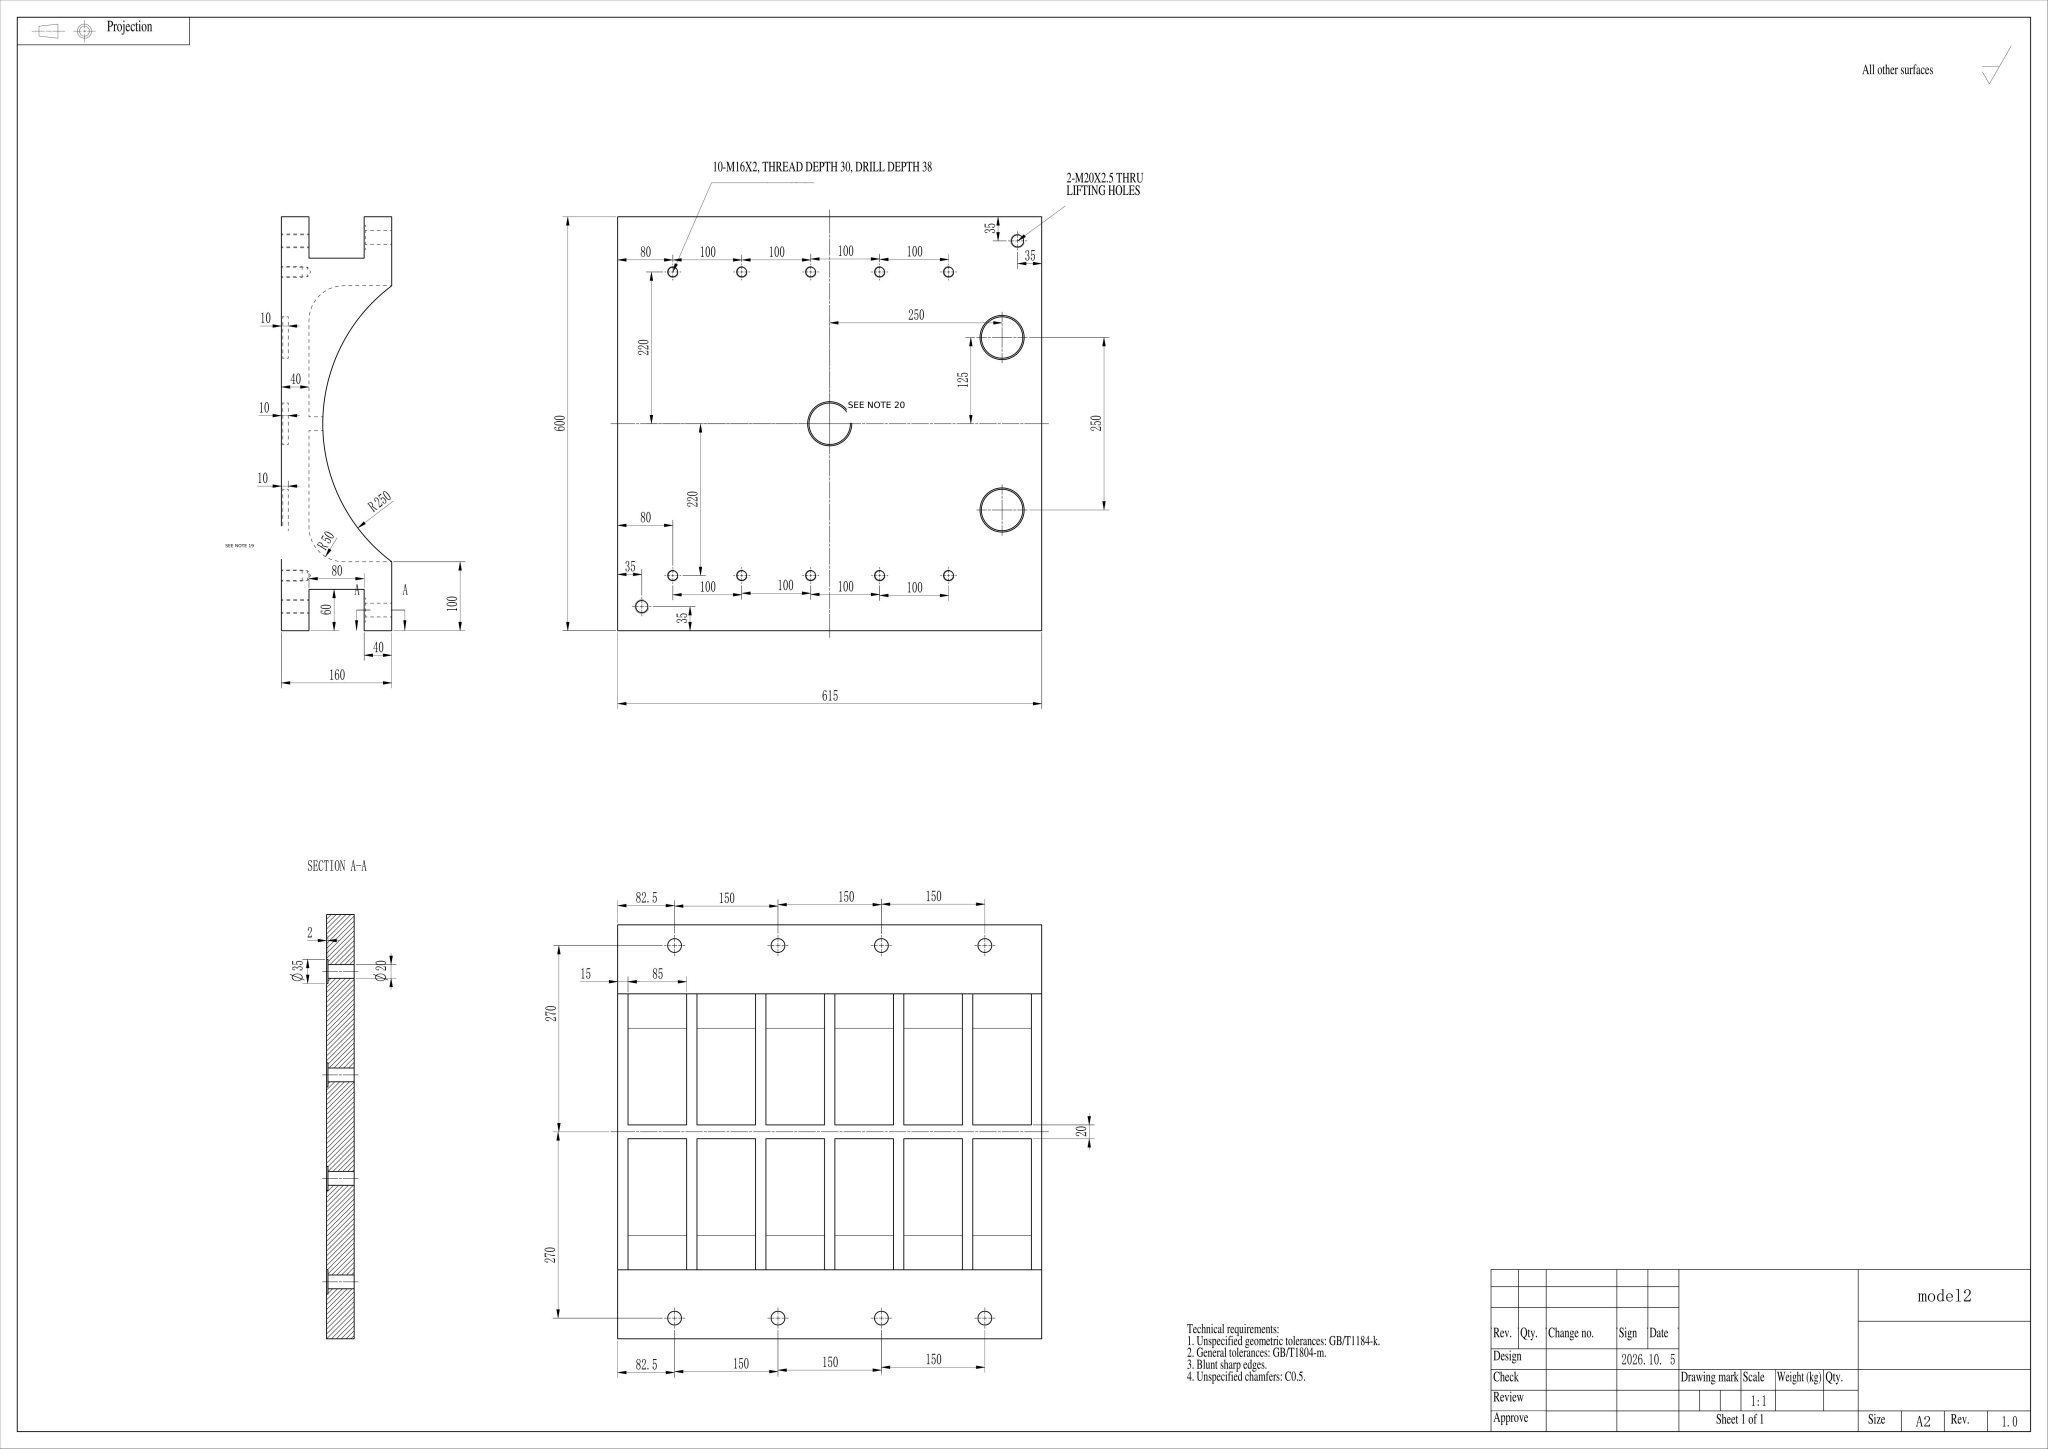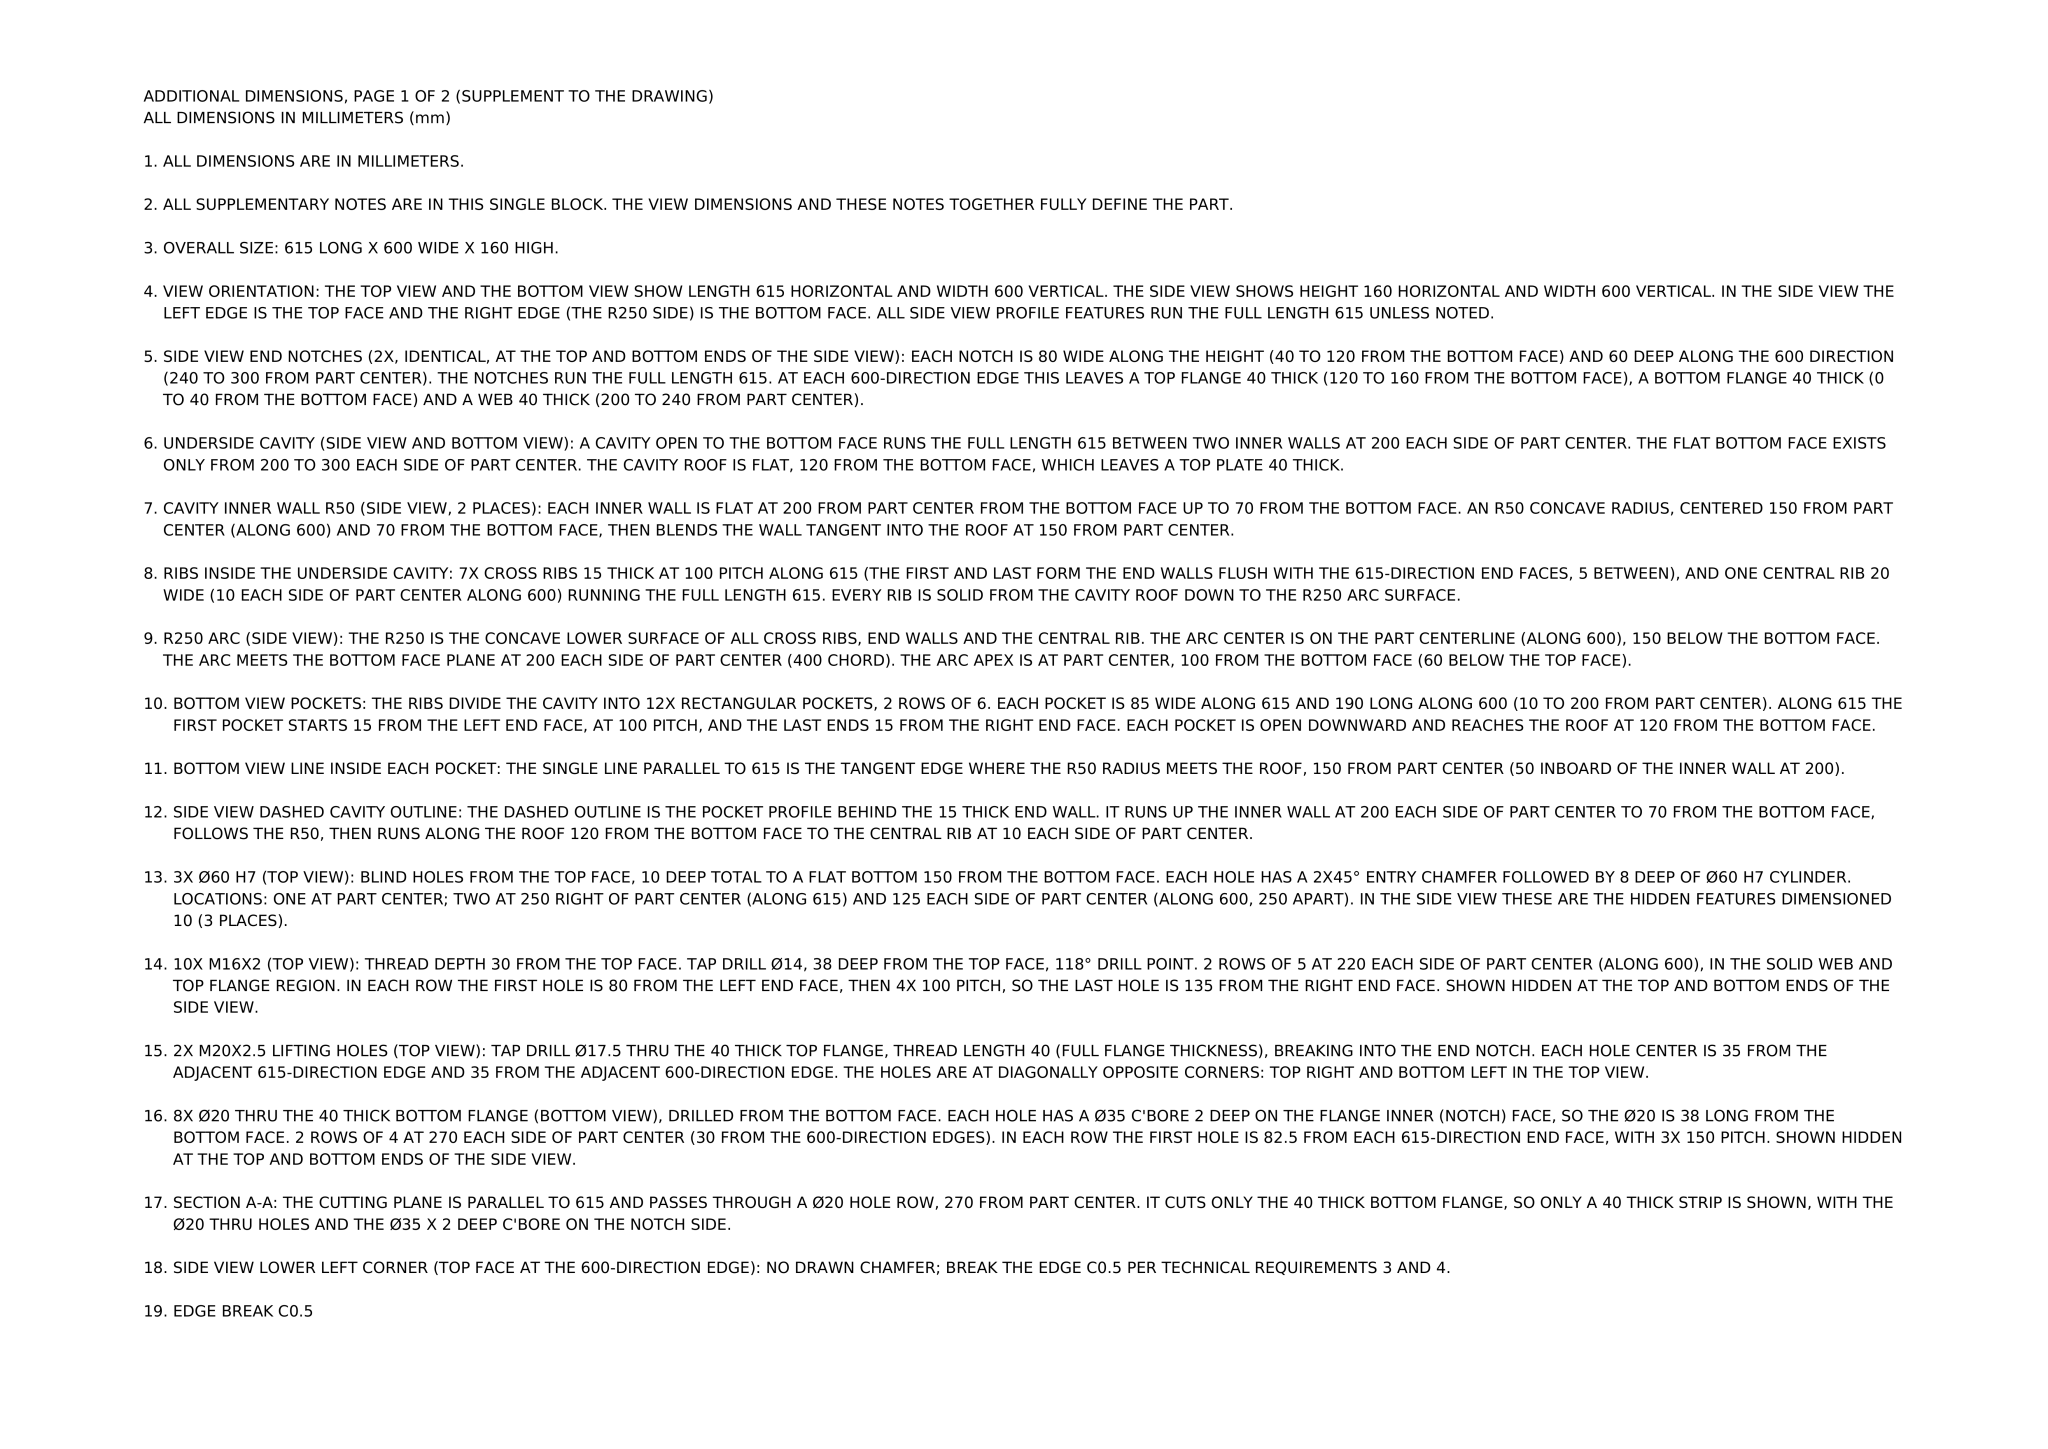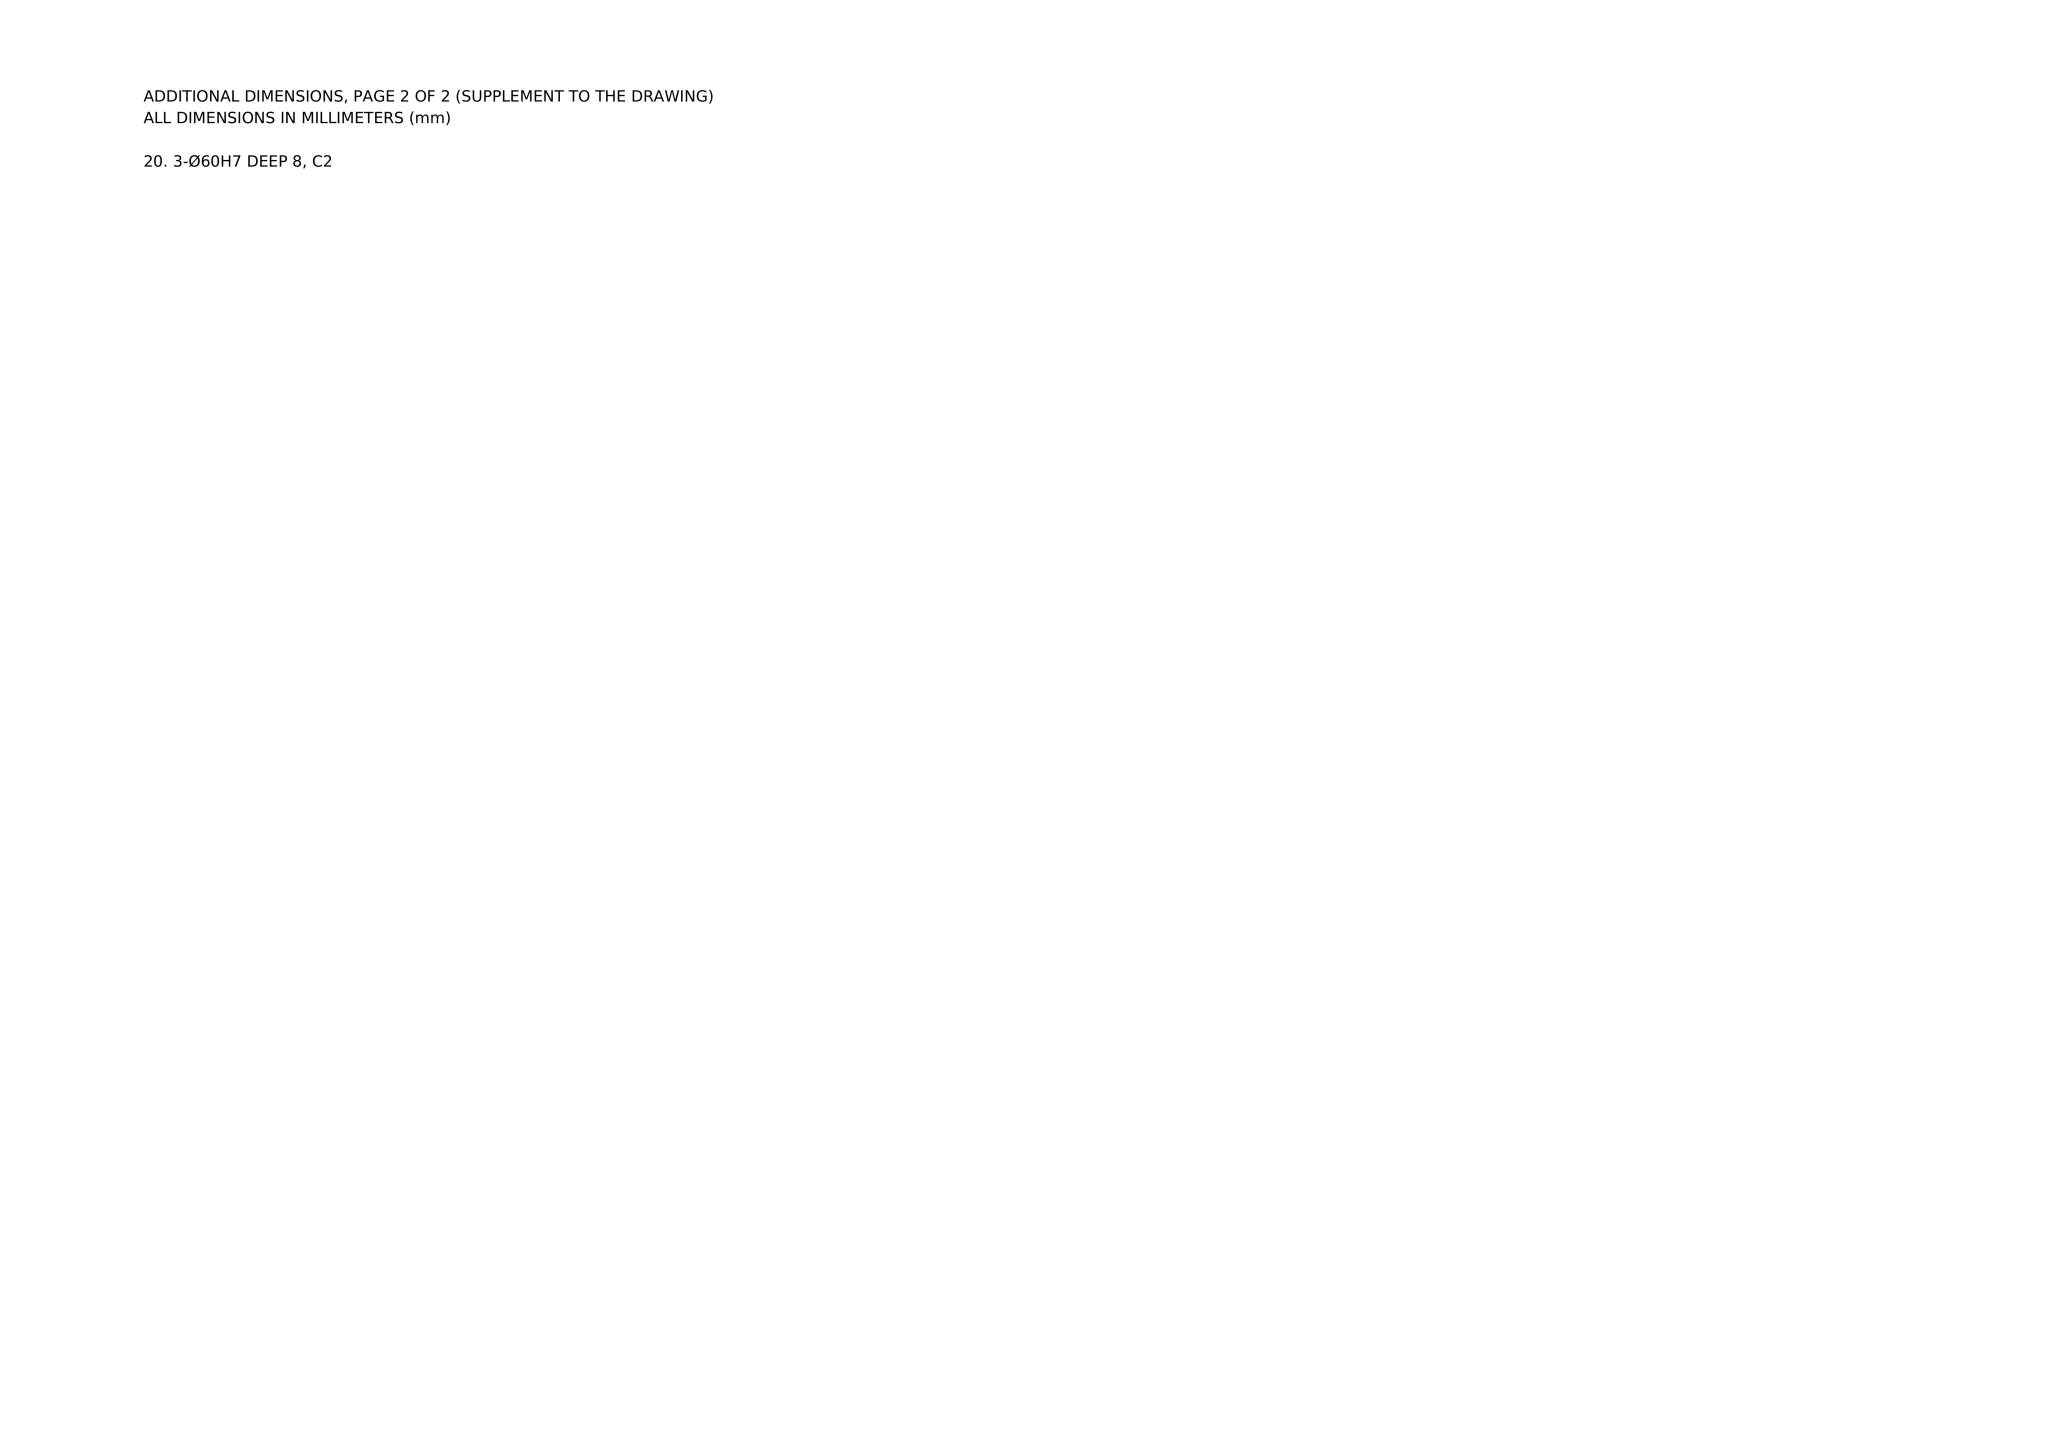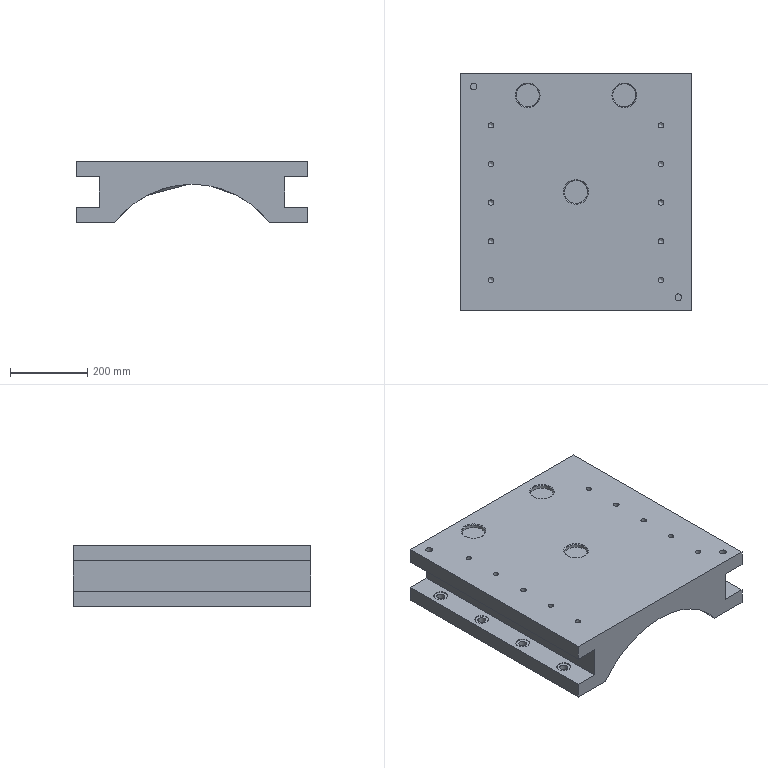Part | NX | mm | 1 solid | 143 faces | box 600 x 615 x 160 mm | volume 26195766 mm3 | plane 86 | cylinder 44 | cone 13 | commonest cylinder face diameters 100 x12 14 x10 20 x8 35 x8 60 x3 17.5 x2 500 x1